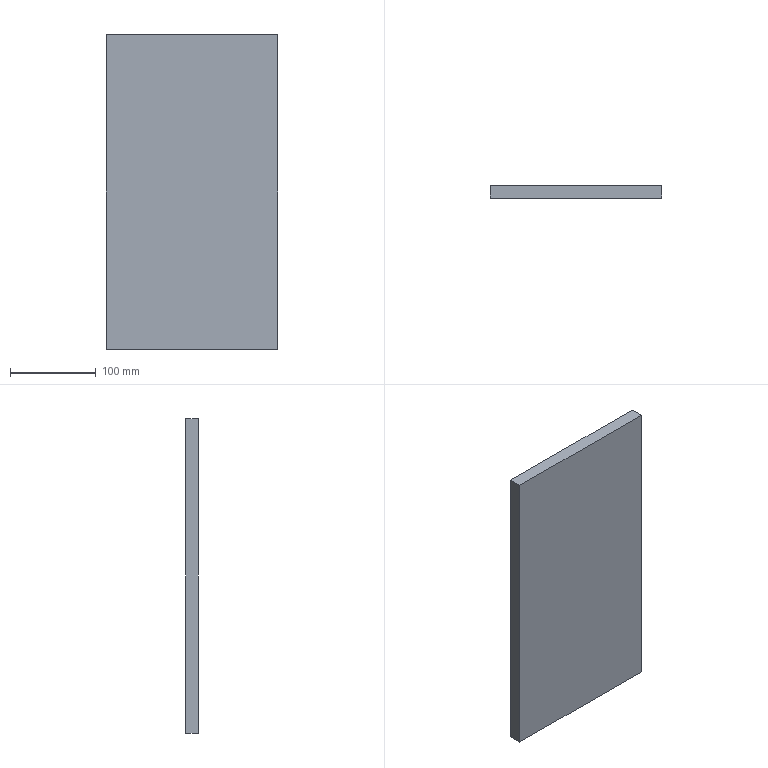Component | SolidWorks | NewDieSet-1_UpperDieSetAssembly-1_MoldUpperPlate510x280-1 | 1 solid | 6 faces | box 200 x 15 x 366 mm | volume 1098000 mm3 | plane 6
build123d program:
from build123d import *

# Parameters (mm, degrees)
SKETCH1_W           = 200
SKETCH1_H           = 366
BOSS_EXTRUDE1_DEPTH = 15


with BuildPart() as part:
    # Sketch1 → Boss-Extrude1 (new body)
    with BuildSketch(Plane.XY):
        with Locations((100, 183)):
            Rectangle(SKETCH1_W, SKETCH1_H)
    extrude(amount=BOSS_EXTRUDE1_DEPTH)


solid = part.part

# Placed as in the assembly
solid = solid.moved(Location((-156.746, 95.927, 170), (90, 0, 0)))
STEP:
#1=CARTESIAN_POINT('',(-6.171,3.186,6.693));
#2=VERTEX_POINT('',#1);
#3=CARTESIAN_POINT('',(-6.171,3.186,21.102));
#4=VERTEX_POINT('',#3);
#5=CARTESIAN_POINT('',(-6.171,3.186,21.102));
#6=DIRECTION('',(0.,0.,1.));
#7=VECTOR('',#6,39.37);
#8=LINE('',#5,#7);
#9=EDGE_CURVE('',#2,#4,#8,.T.);
#10=ORIENTED_EDGE('',*,*,#9,.T.);
#11=CARTESIAN_POINT('',(-6.171,3.777,21.102));
#12=VERTEX_POINT('',#11);
#13=CARTESIAN_POINT('',(-6.171,3.777,21.102));
#14=DIRECTION('',(0.,-1.,0.));
#15=VECTOR('',#14,39.37);
#16=LINE('',#13,#15);
#17=EDGE_CURVE('',#12,#4,#16,.T.);
#18=ORIENTED_EDGE('',*,*,#17,.F.);
#19=CARTESIAN_POINT('',(-6.171,3.777,6.693));
#20=VERTEX_POINT('',#19);
#21=CARTESIAN_POINT('',(-6.171,3.777,21.102));
#22=DIRECTION('',(0.,0.,1.));
#23=VECTOR('',#22,39.37);
#24=LINE('',#21,#23);
#25=EDGE_CURVE('',#20,#12,#24,.T.);
#26=ORIENTED_EDGE('',*,*,#25,.F.);
#27=CARTESIAN_POINT('',(-6.171,3.777,6.693));
#28=DIRECTION('',(0.,-1.,0.));
#29=VECTOR('',#28,39.37);
#30=LINE('',#27,#29);
#31=EDGE_CURVE('',#20,#2,#30,.T.);
#32=ORIENTED_EDGE('',*,*,#31,.T.);
#33=EDGE_LOOP('',(#10,#18,#26,#32));
#34=FACE_OUTER_BOUND('',#33,.T.);
#35=CARTESIAN_POINT('',(-6.171,3.777,21.102));
#36=DIRECTION('',(1.,0.,0.));
#37=DIRECTION('',(0.,-1.,0.));
#38=AXIS2_PLACEMENT_3D('',#35,#36,#37);
#39=PLANE('',#38);
#40=ADVANCED_FACE('',(#34),#39,.F.);
#41=CARTESIAN_POINT('',(1.703,3.186,21.102));
#42=VERTEX_POINT('',#41);
#43=CARTESIAN_POINT('',(-6.171,3.186,21.102));
#44=DIRECTION('',(1.,0.,0.));
#45=VECTOR('',#44,39.37);
#46=LINE('',#43,#45);
#47=EDGE_CURVE('',#4,#42,#46,.T.);
#48=ORIENTED_EDGE('',*,*,#47,.T.);
#49=CARTESIAN_POINT('',(1.703,3.777,21.102));
#50=VERTEX_POINT('',#49);
#51=CARTESIAN_POINT('',(1.703,3.777,21.102));
#52=DIRECTION('',(0.,-1.,0.));
#53=VECTOR('',#52,39.37);
#54=LINE('',#51,#53);
#55=EDGE_CURVE('',#50,#42,#54,.T.);
#56=ORIENTED_EDGE('',*,*,#55,.F.);
#57=CARTESIAN_POINT('',(-6.171,3.777,21.102));
#58=DIRECTION('',(1.,0.,0.));
#59=VECTOR('',#58,39.37);
#60=LINE('',#57,#59);
#61=EDGE_CURVE('',#12,#50,#60,.T.);
#62=ORIENTED_EDGE('',*,*,#61,.F.);
#63=ORIENTED_EDGE('',*,*,#17,.T.);
#64=EDGE_LOOP('',(#48,#56,#62,#63));
#65=FACE_OUTER_BOUND('',#64,.T.);
#66=CARTESIAN_POINT('',(-6.171,3.777,21.102));
#67=DIRECTION('',(0.,0.,-1.));
#68=DIRECTION('',(0.,1.,0.));
#69=AXIS2_PLACEMENT_3D('',#66,#67,#68);
#70=PLANE('',#69);
#71=ADVANCED_FACE('',(#65),#70,.F.);
#72=CARTESIAN_POINT('',(1.703,3.186,6.693));
#73=VERTEX_POINT('',#72);
#74=CARTESIAN_POINT('',(1.703,3.186,21.102));
#75=DIRECTION('',(0.,0.,-1.));
#76=VECTOR('',#75,39.37);
#77=LINE('',#74,#76);
#78=EDGE_CURVE('',#42,#73,#77,.T.);
#79=ORIENTED_EDGE('',*,*,#78,.T.);
#80=CARTESIAN_POINT('',(1.703,3.777,6.693));
#81=VERTEX_POINT('',#80);
#82=CARTESIAN_POINT('',(1.703,3.777,6.693));
#83=DIRECTION('',(0.,-1.,0.));
#84=VECTOR('',#83,39.37);
#85=LINE('',#82,#84);
#86=EDGE_CURVE('',#81,#73,#85,.T.);
#87=ORIENTED_EDGE('',*,*,#86,.F.);
#88=CARTESIAN_POINT('',(1.703,3.777,21.102));
#89=DIRECTION('',(0.,0.,-1.));
#90=VECTOR('',#89,39.37);
#91=LINE('',#88,#90);
#92=EDGE_CURVE('',#50,#81,#91,.T.);
#93=ORIENTED_EDGE('',*,*,#92,.F.);
#94=ORIENTED_EDGE('',*,*,#55,.T.);
#95=EDGE_LOOP('',(#79,#87,#93,#94));
#96=FACE_OUTER_BOUND('',#95,.T.);
#97=CARTESIAN_POINT('',(1.703,3.777,21.102));
#98=DIRECTION('',(-1.,0.,0.));
#99=DIRECTION('',(0.,1.,0.));
#100=AXIS2_PLACEMENT_3D('',#97,#98,#99);
#101=PLANE('',#100);
#102=ADVANCED_FACE('',(#96),#101,.F.);
#103=CARTESIAN_POINT('',(-6.171,3.186,6.693));
#104=DIRECTION('',(-1.,0.,0.));
#105=VECTOR('',#104,39.37);
#106=LINE('',#103,#105);
#107=EDGE_CURVE('',#73,#2,#106,.T.);
#108=ORIENTED_EDGE('',*,*,#107,.T.);
#109=ORIENTED_EDGE('',*,*,#31,.F.);
#110=CARTESIAN_POINT('',(-6.171,3.777,6.693));
#111=DIRECTION('',(-1.,0.,0.));
#112=VECTOR('',#111,39.37);
#113=LINE('',#110,#112);
#114=EDGE_CURVE('',#81,#20,#113,.T.);
#115=ORIENTED_EDGE('',*,*,#114,.F.);
#116=ORIENTED_EDGE('',*,*,#86,.T.);
#117=EDGE_LOOP('',(#108,#109,#115,#116));
#118=FACE_OUTER_BOUND('',#117,.T.);
#119=CARTESIAN_POINT('',(-6.171,3.777,6.693));
#120=DIRECTION('',(0.,0.,1.));
#121=DIRECTION('',(0.,-1.,0.));
#122=AXIS2_PLACEMENT_3D('',#119,#120,#121);
#123=PLANE('',#122);
#124=ADVANCED_FACE('',(#118),#123,.F.);
#125=ORIENTED_EDGE('',*,*,#25,.T.);
#126=ORIENTED_EDGE('',*,*,#61,.T.);
#127=ORIENTED_EDGE('',*,*,#92,.T.);
#128=ORIENTED_EDGE('',*,*,#114,.T.);
#129=EDGE_LOOP('',(#125,#126,#127,#128));
#130=FACE_OUTER_BOUND('',#129,.T.);
#131=CARTESIAN_POINT('',(-6.171,3.777,21.102));
#132=DIRECTION('',(0.,-1.,0.));
#133=DIRECTION('',(-1.,0.,0.));
#134=AXIS2_PLACEMENT_3D('',#131,#132,#133);
#135=PLANE('',#134);
#136=ADVANCED_FACE('',(#130),#135,.F.);
#137=ORIENTED_EDGE('',*,*,#9,.F.);
#138=ORIENTED_EDGE('',*,*,#107,.F.);
#139=ORIENTED_EDGE('',*,*,#78,.F.);
#140=ORIENTED_EDGE('',*,*,#47,.F.);
#141=EDGE_LOOP('',(#137,#138,#139,#140));
#142=FACE_OUTER_BOUND('',#141,.T.);
#143=CARTESIAN_POINT('',(-6.171,3.186,21.102));
#144=DIRECTION('',(0.,-1.,0.));
#145=DIRECTION('',(-1.,0.,0.));
#146=AXIS2_PLACEMENT_3D('',#143,#144,#145);
#147=PLANE('',#146);
#148=ADVANCED_FACE('',(#142),#147,.T.);
#149=CLOSED_SHELL('',(#40,#71,#102,#124,#136,#148));
#150=MANIFOLD_SOLID_BREP('',#149);
#151=CARTESIAN_POINT('',(0.,0.,0.));
#152=DIRECTION('',(0.,0.,1.));
#153=DIRECTION('',(1.,0.,0.));
#154=AXIS2_PLACEMENT_3D('',#151,#152,#153);
#155=(LENGTH_UNIT()NAMED_UNIT(*)SI_UNIT($,.METRE.));
#156=LENGTH_MEASURE_WITH_UNIT(LENGTH_MEASURE(0.0254),#155);
#157=DIMENSIONAL_EXPONENTS(1.,0.,0.,0.,0.,0.,0.);
#158=(CONVERSION_BASED_UNIT('',#156)LENGTH_UNIT()NAMED_UNIT(#157));
#159=UNCERTAINTY_MEASURE_WITH_UNIT(LENGTH_MEASURE(0.00001),#158,'','');
#160=(NAMED_UNIT(*)PLANE_ANGLE_UNIT()SI_UNIT($,.RADIAN.));
#161=(NAMED_UNIT(*)SI_UNIT($,.STERADIAN.)SOLID_ANGLE_UNIT());
#162=(GEOMETRIC_REPRESENTATION_CONTEXT(3)GLOBAL_UNCERTAINTY_ASSIGNED_CONTEXT((#159))GLOBAL_UNIT_ASSIGNED_CONTEXT((#158,#160,#161))REPRESENTATION_CONTEXT('',''));
#163=ADVANCED_BREP_SHAPE_REPRESENTATION('',(#150,#154),#162);
#164=COLOUR_RGB('',0.7922,0.8196,0.9333);
#165=FILL_AREA_STYLE_COLOUR('',#164);
#166=FILL_AREA_STYLE('',(#165));
#167=SURFACE_STYLE_FILL_AREA(#166);
#168=SURFACE_SIDE_STYLE('',(#167));
#169=SURFACE_STYLE_USAGE(.BOTH.,#168);
#170=PRESENTATION_STYLE_ASSIGNMENT((#169));
#171=STYLED_ITEM('',(#170),#150);
#172=(LENGTH_UNIT()NAMED_UNIT(*)SI_UNIT($,.METRE.));
#173=LENGTH_MEASURE_WITH_UNIT(LENGTH_MEASURE(0.0254),#172);
#174=DIMENSIONAL_EXPONENTS(1.,0.,0.,0.,0.,0.,0.);
#175=(CONVERSION_BASED_UNIT('',#173)LENGTH_UNIT()NAMED_UNIT(#174));
#176=UNCERTAINTY_MEASURE_WITH_UNIT(LENGTH_MEASURE(0.00001),#175,'','');
#177=(NAMED_UNIT(*)PLANE_ANGLE_UNIT()SI_UNIT($,.RADIAN.));
#178=(NAMED_UNIT(*)SI_UNIT($,.STERADIAN.)SOLID_ANGLE_UNIT());
#179=(GEOMETRIC_REPRESENTATION_CONTEXT(3)GLOBAL_UNCERTAINTY_ASSIGNED_CONTEXT((#176))GLOBAL_UNIT_ASSIGNED_CONTEXT((#175,#177,#178))REPRESENTATION_CONTEXT('',''));
#180=MECHANICAL_DESIGN_GEOMETRIC_PRESENTATION_REPRESENTATION('',(#171),#179);
#181=PRESENTATION_LAYER_ASSIGNMENT('','',(#171));